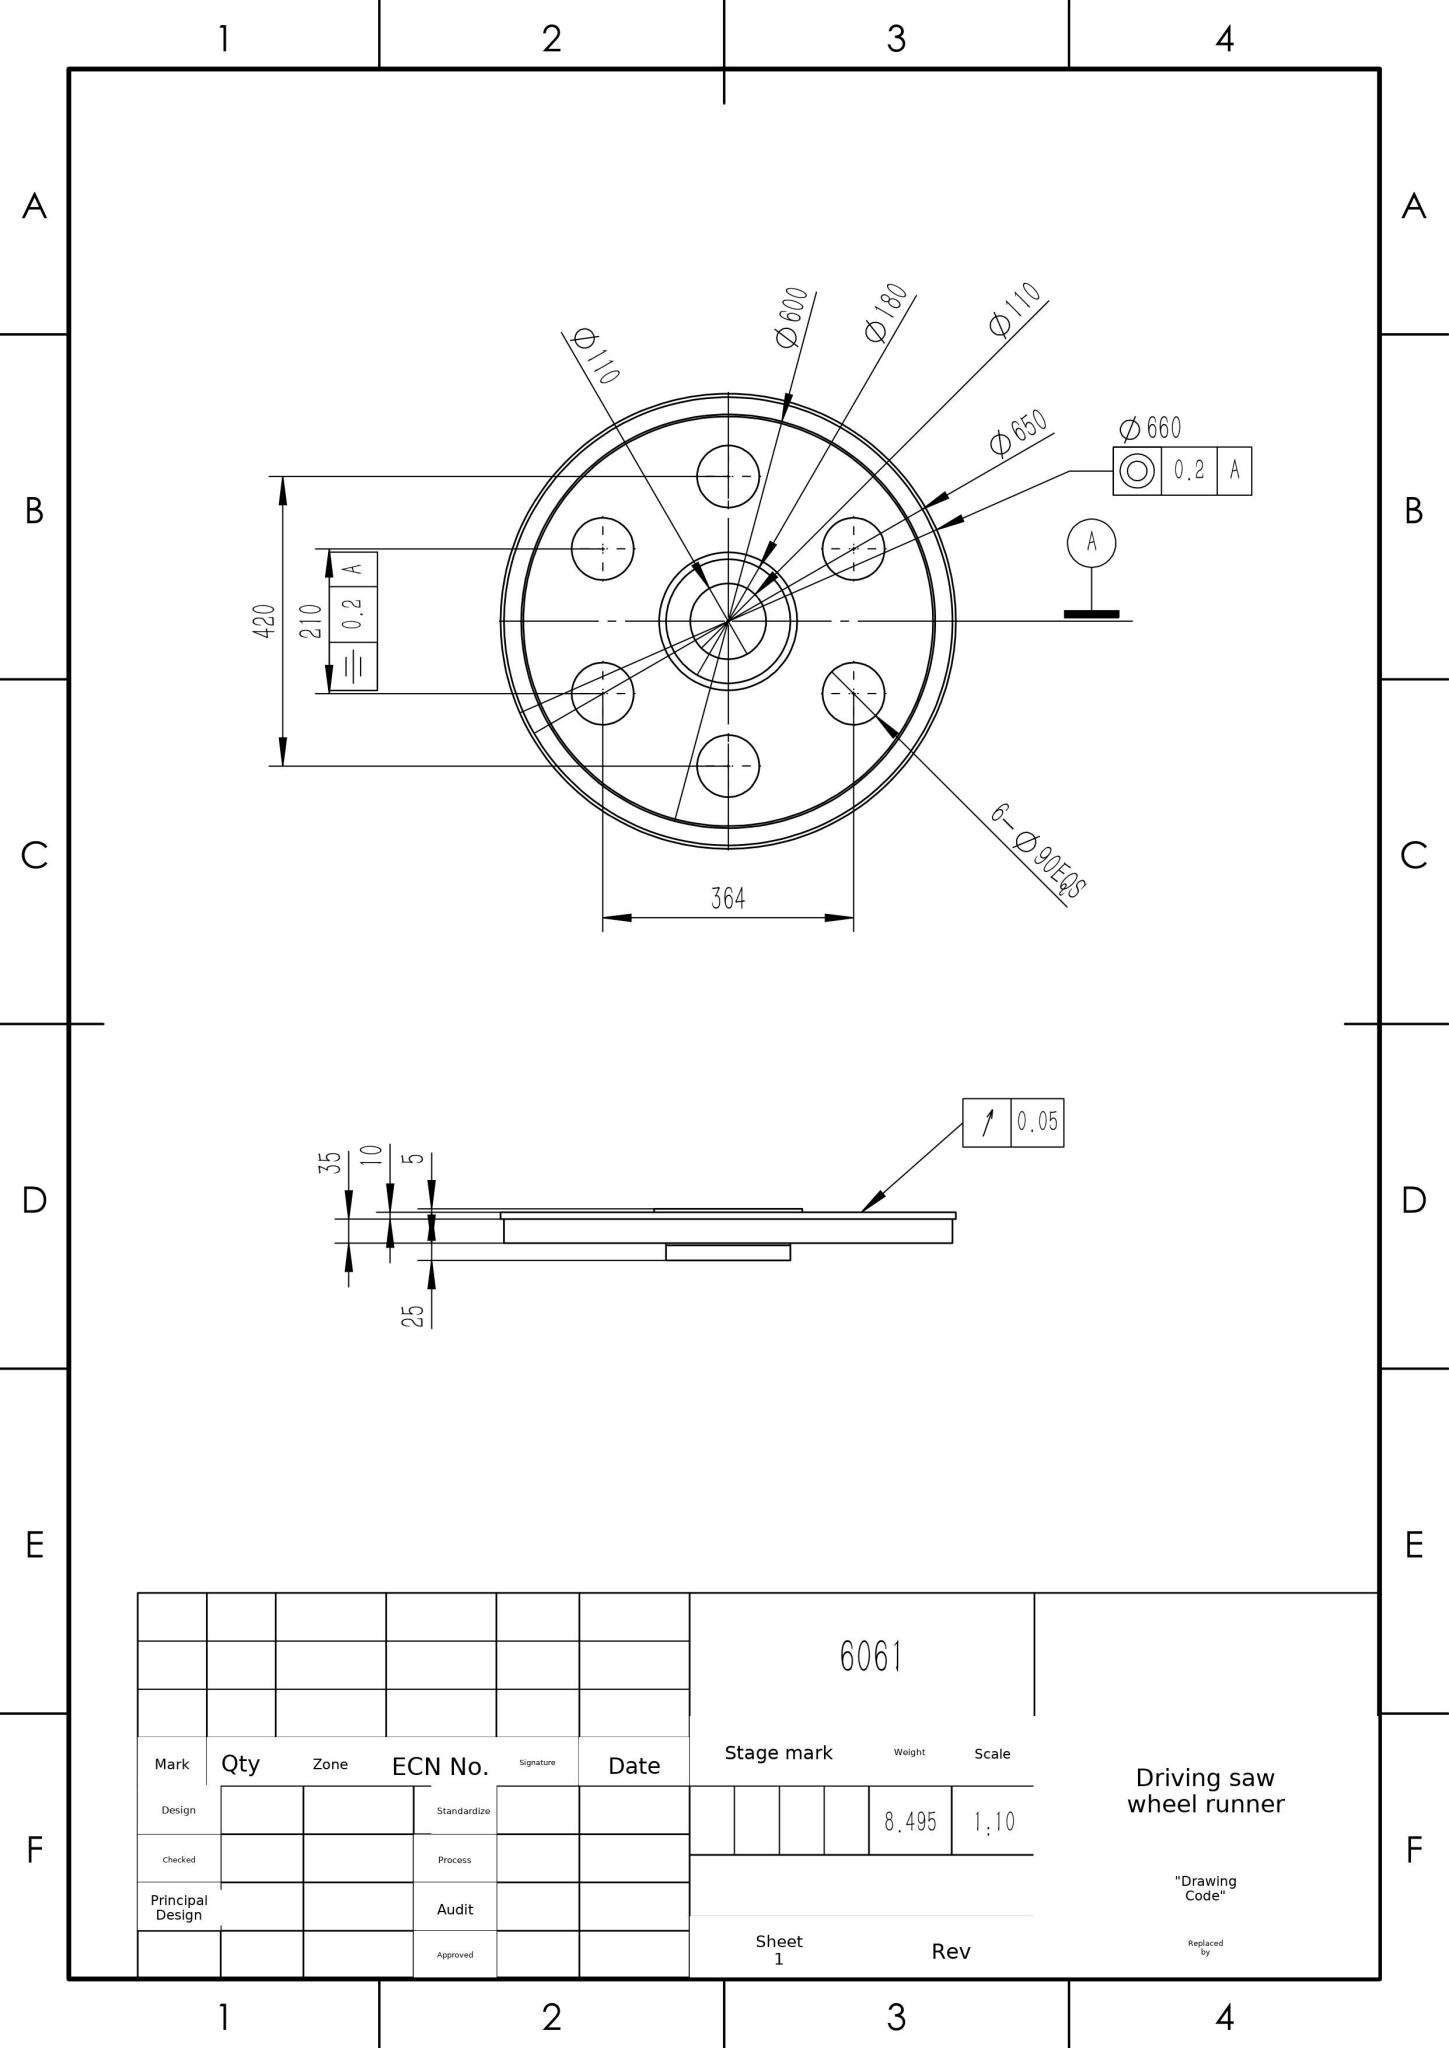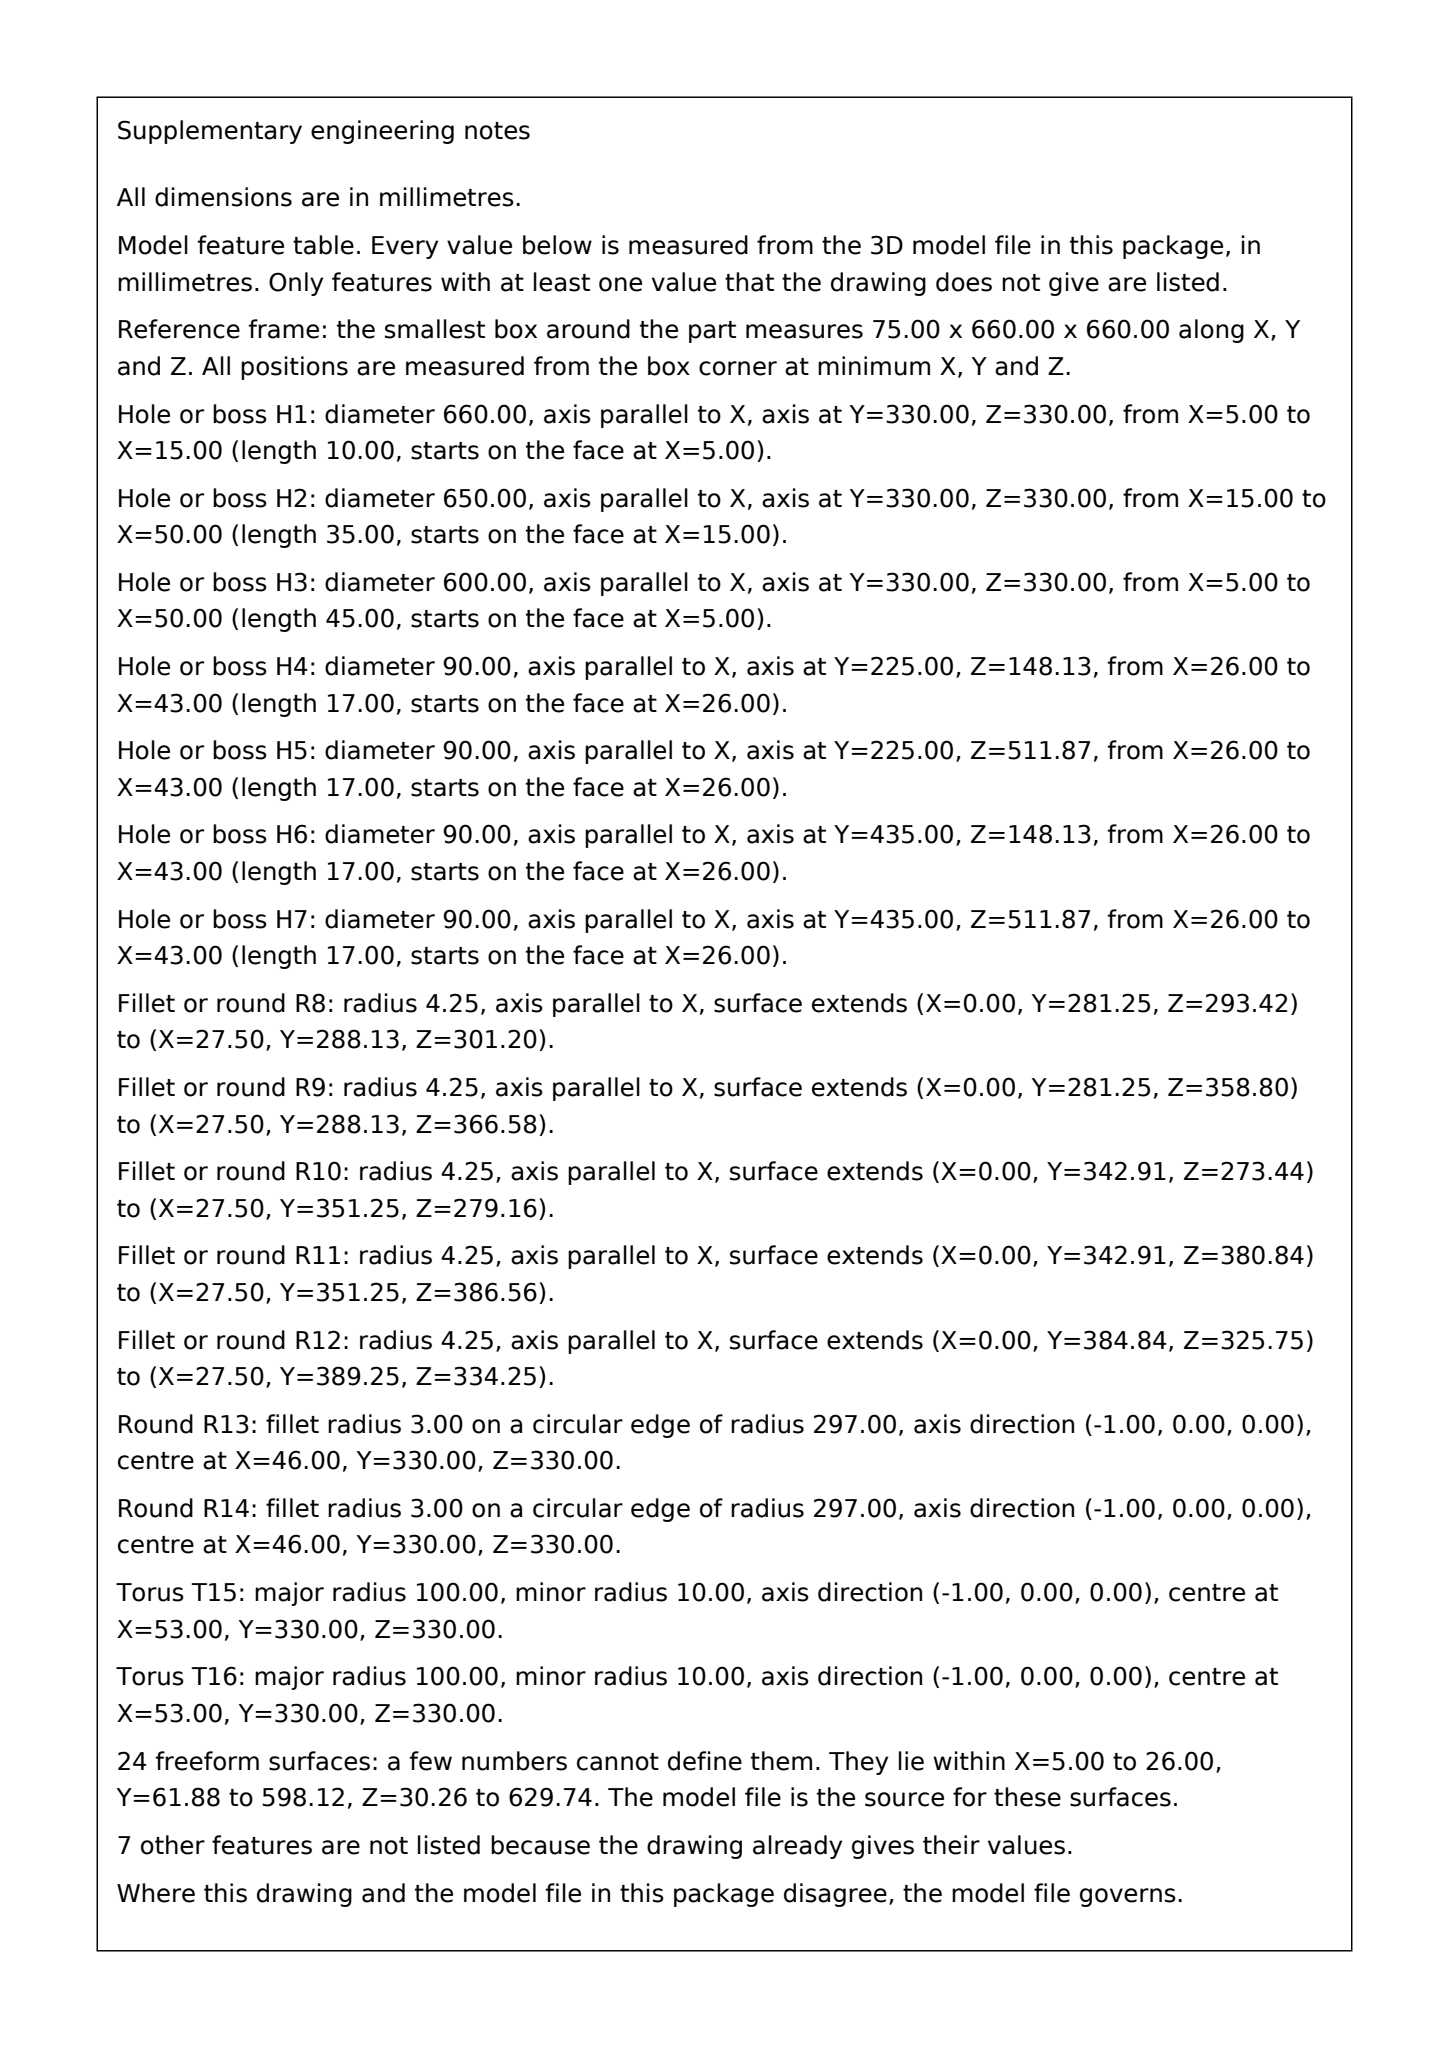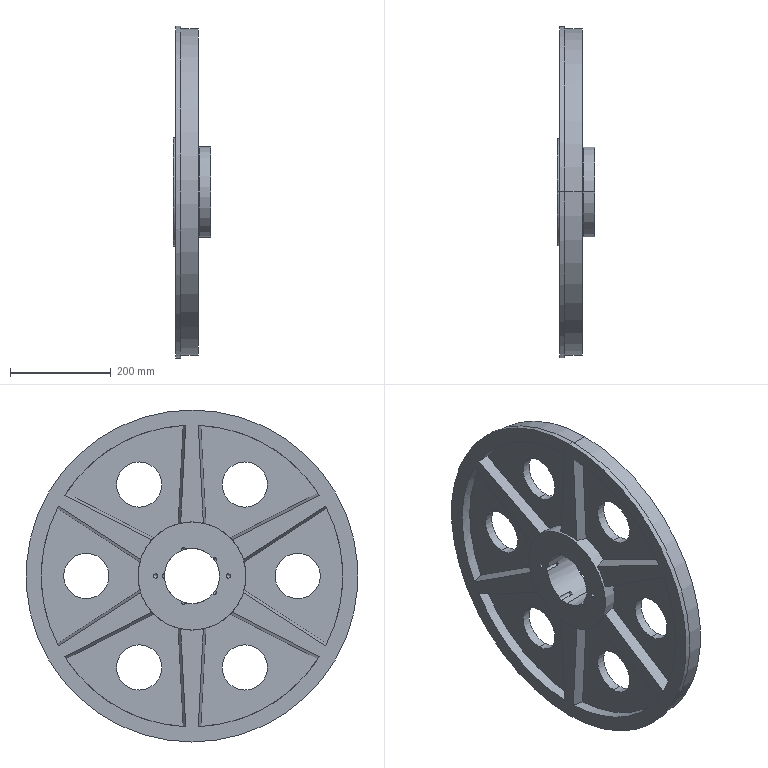Part | SolidWorks | mm | material 6061 | 1 solid | 96 faces | box 75 x 660 x 660 mm | volume 8495500 mm3 | cylinder 43 | spline 24 | cone 13 | plane 12 | torus 4 | commonest cylinder face diameters 8.5 x13 90 x12 600 x8 215 x2 660 x2 650 x2 180 x2 110 x2